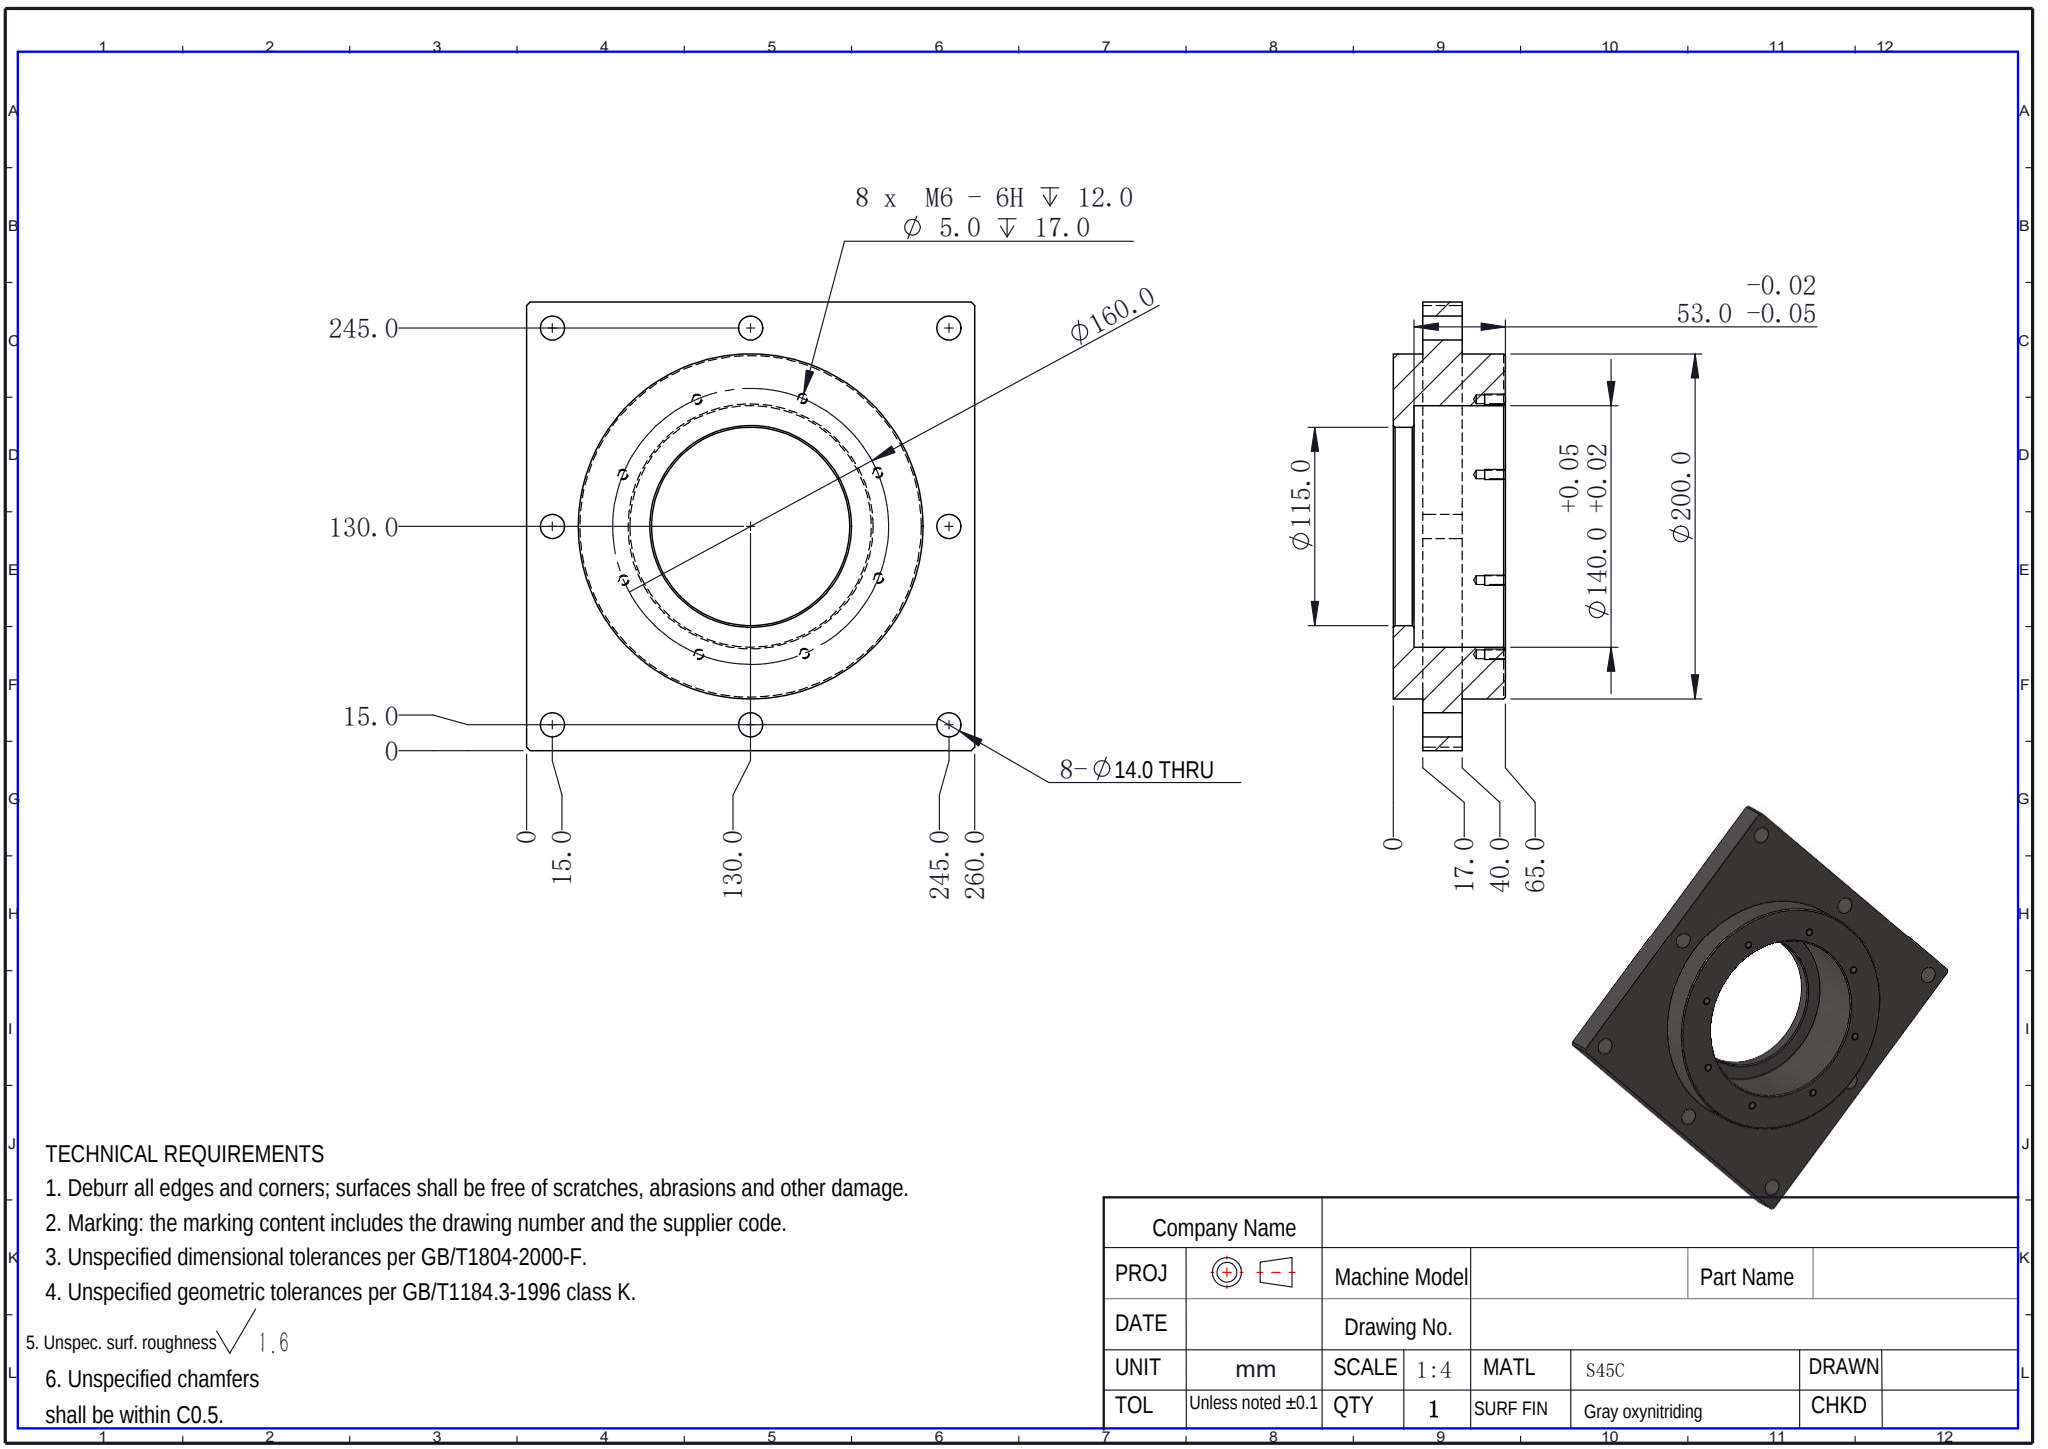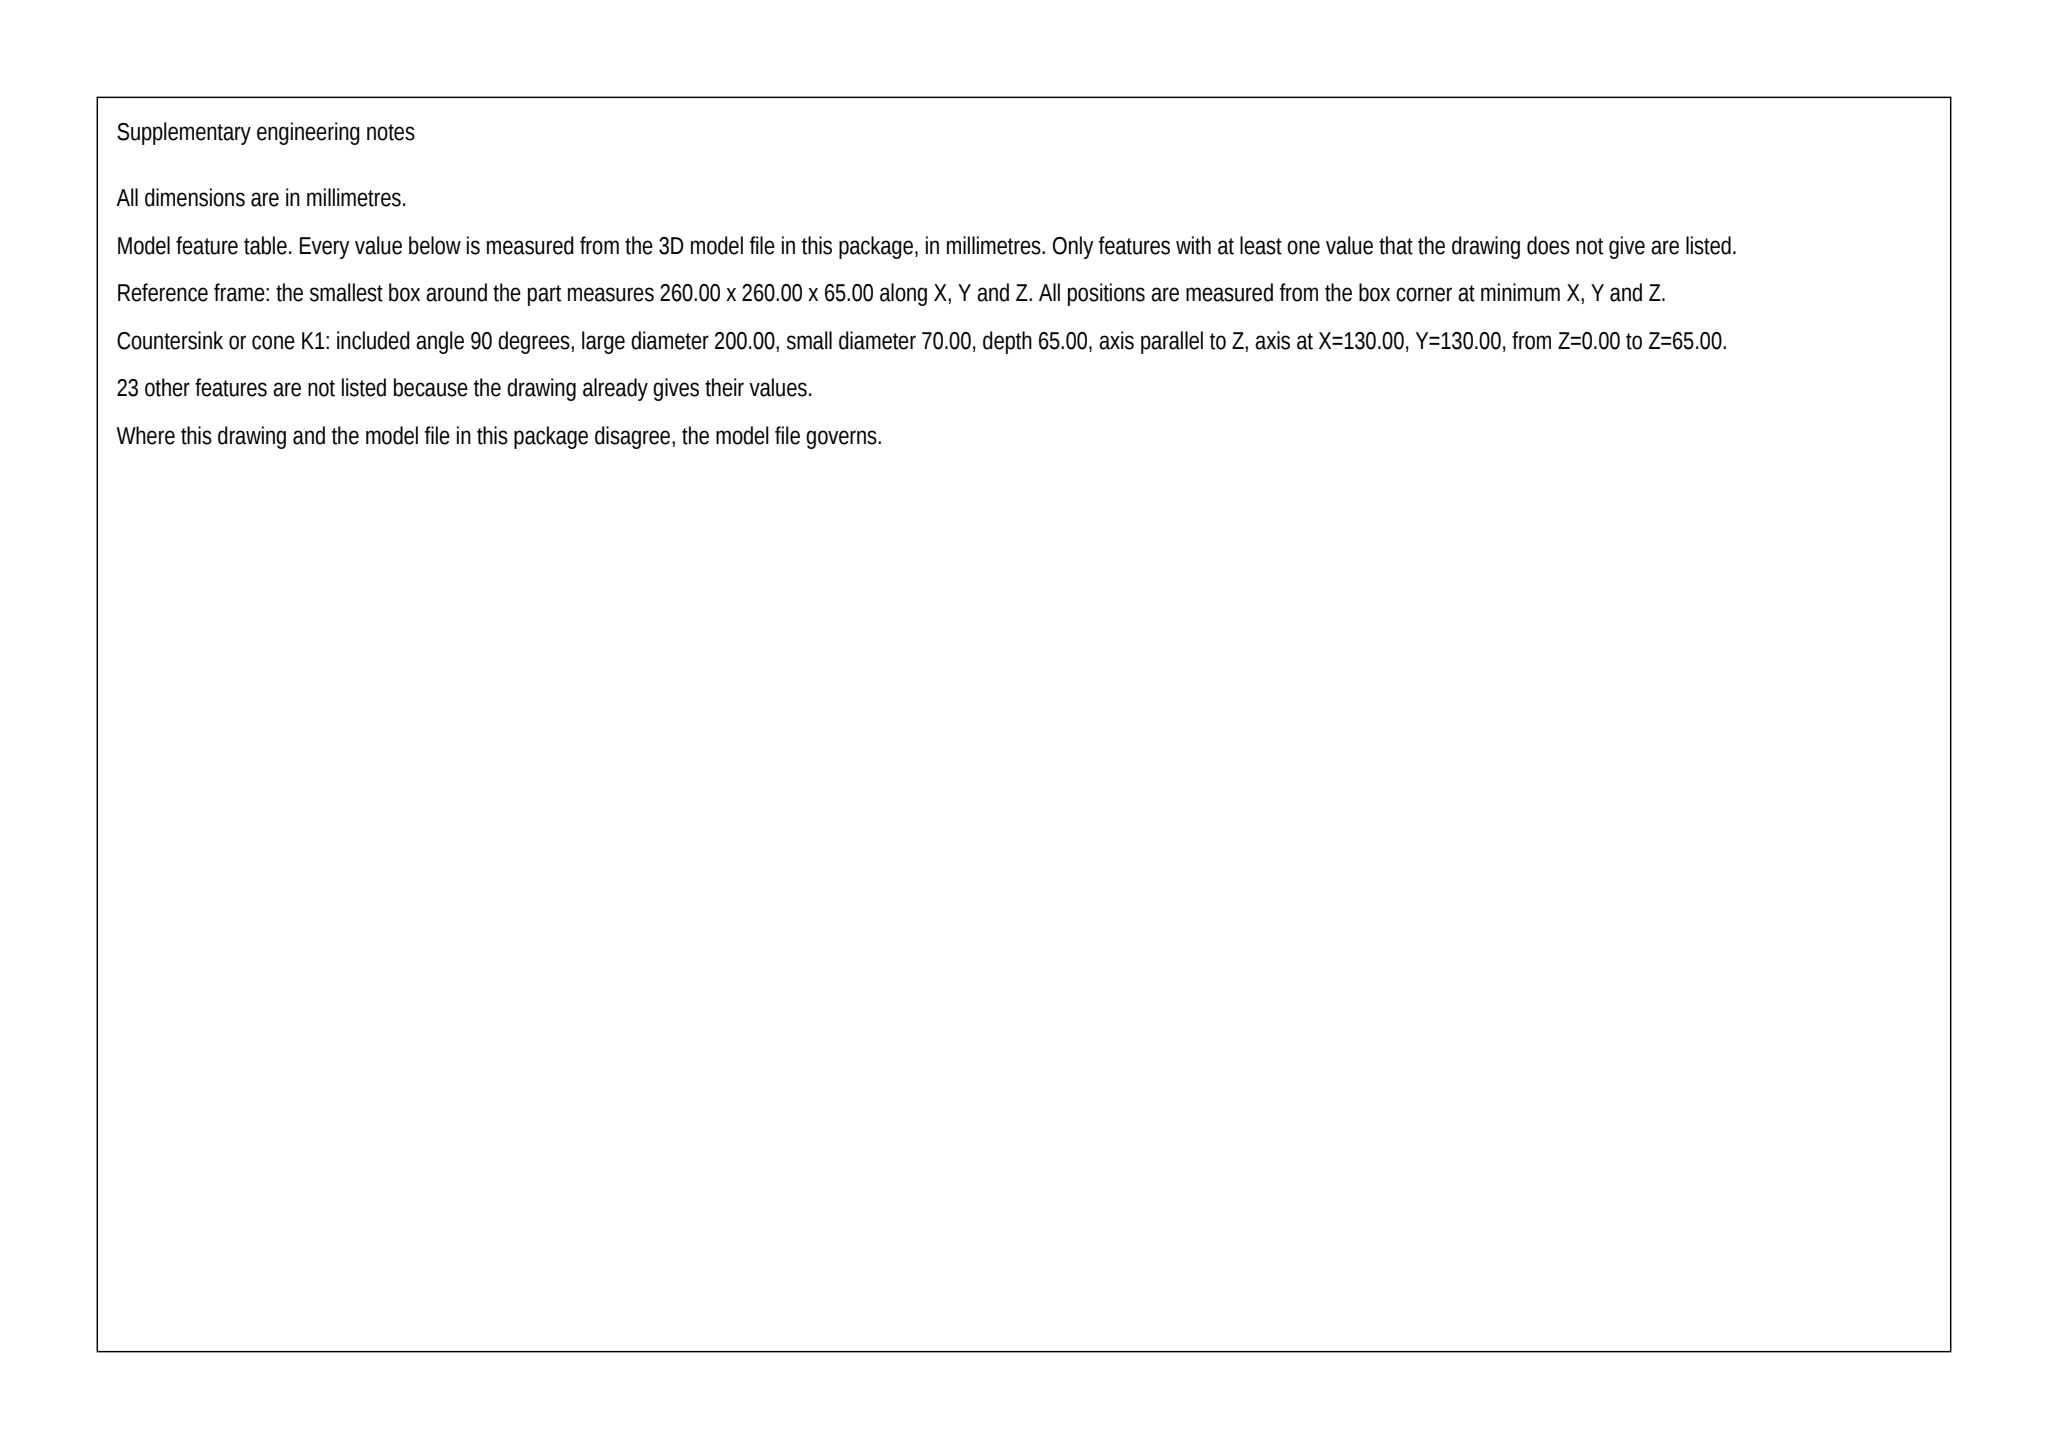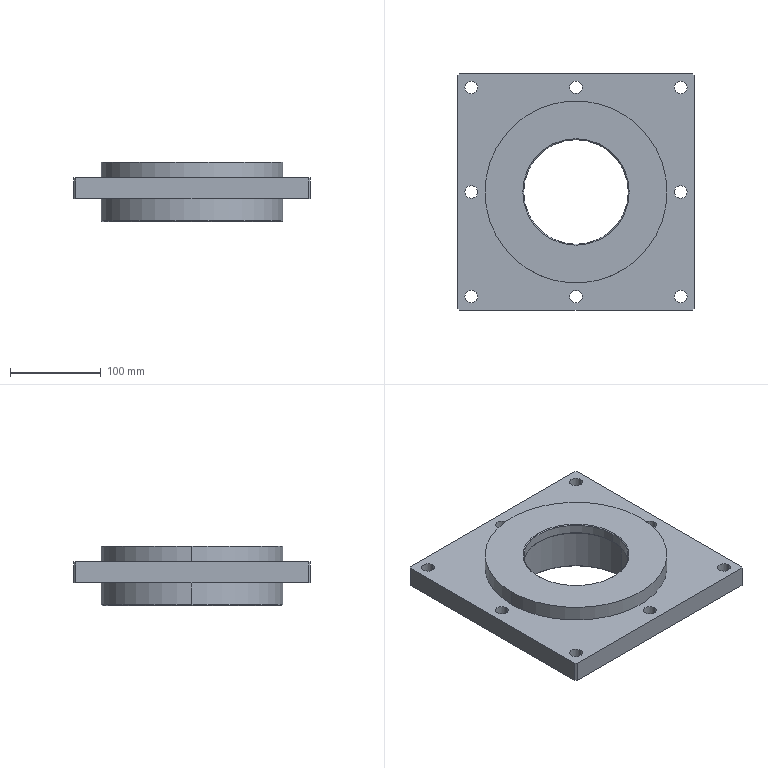Part | SolidWorks | mm | 1 solid | 77 faces | box 260 x 260 x 65 mm | volume 1901600 mm3 | cylinder 40 | cone 24 | plane 13 | commonest cylinder face diameters 5 x16 14 x16 200 x4 140 x2 115 x2
Drawing notes:
PLATE 260.0 SQ; OVERALL Y 260.0 FROM BTM EDGE 0 | from the solid: bbox_xyz [260.0,260.0,65.0]; planes y=0.0 and y=260.0
8X M6 ON Ø160 B.C. EQ SP 45°, 1ST HOLE 22.9° CCW FROM HORIZ CL | from the solid: Ø5 holes at R80 from (130,130): angles 22.92,67.94,112.92,157.94,202.92,247.94,292.92,337.94 deg (45° pitch, 22.93° offset)
build123d program:
from build123d import *

# Parameters (mm, degrees)
SKETCH1_W             = 260
SKETCH1_H             = 260
BOSS_EXTRUDE1_DEPTH   = 11.5
BOSS_EXTRUDE2_START   = 17
SKETCH2_R             = 100
BOSS_EXTRUDE2_DEPTH   = 65
SKETCH3_R             = 57.5
CUT_EXTRUDE1_DEPTH    = 141
SKETCH4_R             = 70
CUT_EXTRUDE2_DEPTH    = 53
SKETCH5_R             = 7
CUT_EXTRUDE3_DEPTH    = 46
M6_TAPPED_HOLE1_D     = 5
M6_TAPPED_HOLE1_DEPTH = 17
M6_TAPPED_HOLE1_TIP   = 1.502
CHAMFER1_SIZE         = 2
CHAMFER2_SIZE         = 1


with BuildPart() as part:
    # Sketch1 → Boss-Extrude1 (new, symmetric)
    with BuildSketch(Plane.XY):
        Rectangle(SKETCH1_W, SKETCH1_H)
    extrude(amount=BOSS_EXTRUDE1_DEPTH, both=True)

    # Sketch2 → Boss-Extrude2 (add)
    with BuildSketch(Plane.XY.offset(11.5).offset(BOSS_EXTRUDE2_START)):
        Circle(SKETCH2_R)
    extrude(amount=-BOSS_EXTRUDE2_DEPTH)

    # Sketch3 → Cut-Extrude1 (cut)
    with BuildSketch(Plane(origin=(0, 0, -36.5), x_dir=(-1, 0, 0), z_dir=(0, 0, -1))):
        Circle(SKETCH3_R)
    extrude(amount=-CUT_EXTRUDE1_DEPTH, mode=Mode.SUBTRACT)

    # Sketch4 → Cut-Extrude2 (cut)
    with BuildSketch(Plane(origin=(0, 0, -36.5), x_dir=(-1, 0, 0), z_dir=(0, 0, -1))):
        Circle(SKETCH4_R)
    extrude(amount=-CUT_EXTRUDE2_DEPTH, mode=Mode.SUBTRACT)

    # Sketch5 → Cut-Extrude3 (cut)
    with BuildSketch(Plane.XY.offset(11.5)):
        with Locations((-115, 115)):
            Circle(SKETCH5_R)
        with Locations((0, 115)):
            Circle(SKETCH5_R)
        with Locations((115, 115)):
            Circle(SKETCH5_R)
        with Locations((-115, 0)):
            Circle(SKETCH5_R)
        with Locations((115, 0)):
            Circle(SKETCH5_R)
        with Locations((-115, -115)):
            Circle(SKETCH5_R)
        with Locations((115, -115)):
            Circle(SKETCH5_R)
        with Locations((0, -115)):
            Circle(SKETCH5_R)
    extrude(amount=-CUT_EXTRUDE3_DEPTH, mode=Mode.SUBTRACT)

    # M6 Tapped Hole1
    with Locations(Plane(origin=(0, 0, -36.5), x_dir=(-1, 0, 0), z_dir=(0, 0, -1))):
        with Locations((-74.136, -30.065), (-73.681, 31.163), (-30.065, 74.136), (31.163, 73.681), (74.136, 30.065), (73.681, -31.163), (30.065, -74.136), (-31.163, -73.681)):
            Hole(M6_TAPPED_HOLE1_D / 2, depth=M6_TAPPED_HOLE1_DEPTH)
            with Locations((0, 0, -(M6_TAPPED_HOLE1_DEPTH + M6_TAPPED_HOLE1_TIP / 2))):  # 118° drill point
                Cone(0, M6_TAPPED_HOLE1_D / 2, M6_TAPPED_HOLE1_TIP, mode=Mode.SUBTRACT)

    # Chamfer1
    chamfer1_edges = [part.edges().sort_by_distance(p)[0] for p in [
        (-130, 130, 0),
        (130, 130, 0),
        (130, -130, 0),
        (-130, -130, 0),
    ]]
    chamfer(chamfer1_edges, length=CHAMFER1_SIZE)

    # Chamfer2
    chamfer2_edges = [part.edges().sort_by_distance(p)[0] for p in [
        (-100, 0, -36.5),
        (57.5, 0, 28.5),
        (70, 0, -36.5),
        (57.5, 0, 16.5),
    ]]
    chamfer(chamfer2_edges, length=CHAMFER2_SIZE)


solid = part.part